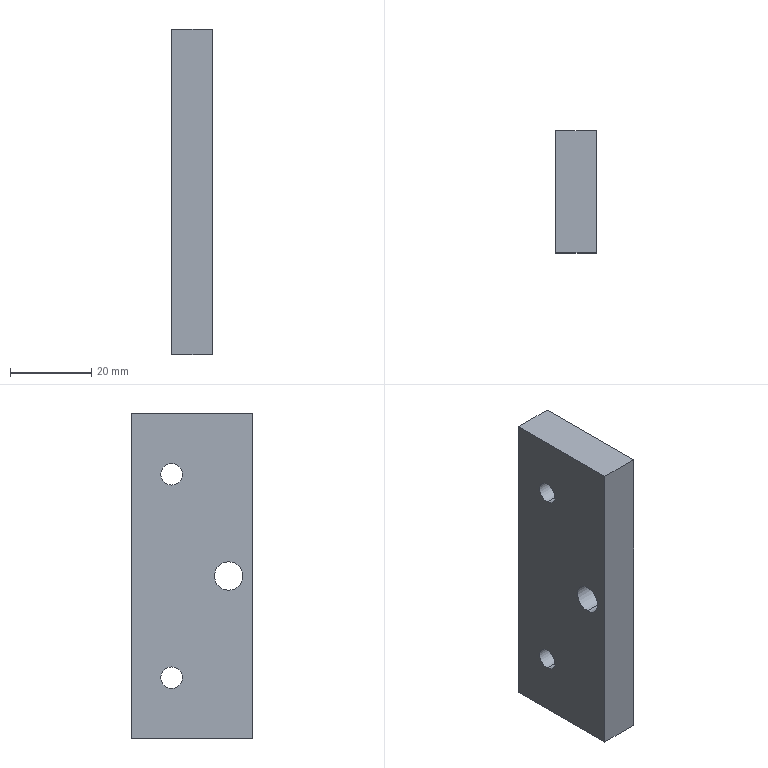Component | SolidWorks | A0131-1 | 1 solid | 18 faces | box 10 x 30 x 80 mm | volume 22564 mm3 | cylinder 10 | plane 8 | commonest cylinder face diameters 10 x4 5.3 x4 7 x2
build123d program:
from build123d import *

# Parameters (mm, degrees)
SKETCH1_W                                       = 80
SKETCH1_H                                       = 30
BOSS_EXTRUDE1_DEPTH                             = 10
M8X1_0_TAPPED_HOLE1_D                           = 7
M5_HEX_SOCKET_HEAD_CAP_SCREW_CBORE1_D           = 5.3
M5_HEX_SOCKET_HEAD_CAP_SCREW_CBORE1_CBORE_D     = 10
M5_HEX_SOCKET_HEAD_CAP_SCREW_CBORE1_CBORE_DEPTH = 5.4


with BuildPart() as part:
    # Sketch1 → Boss-Extrude1 (new body)
    with BuildSketch(Plane.XY):
        Rectangle(SKETCH1_W, SKETCH1_H)
    extrude(amount=BOSS_EXTRUDE1_DEPTH)

    # M8x1.0 Tapped Hole1 (through all)
    with Locations(Plane.XY.offset(10)):
        with Locations((0, 9)):
            Hole(M8X1_0_TAPPED_HOLE1_D / 2)

    # M5 Hex Socket Head Cap Screw CBORE1 (through all)
    with Locations(Plane.XY.offset(10)):
        with Locations((-25, -5), (25, -5)):
            CounterBoreHole(M5_HEX_SOCKET_HEAD_CAP_SCREW_CBORE1_D / 2, M5_HEX_SOCKET_HEAD_CAP_SCREW_CBORE1_CBORE_D / 2, M5_HEX_SOCKET_HEAD_CAP_SCREW_CBORE1_CBORE_DEPTH)


solid = part.part

# Placed as in the assembly
solid = solid.moved(Location((-38.619, 56, 60), (180, 90, 0)))
STEP:
#1=COLOUR_RGB('',0.7922,0.8196,0.9333);
#2=FILL_AREA_STYLE_COLOUR('',#1);
#3=FILL_AREA_STYLE('',(#2));
#4=SURFACE_STYLE_FILL_AREA(#3);
#5=SURFACE_SIDE_STYLE('',(#4));
#6=SURFACE_STYLE_USAGE(.BOTH.,#5);
#7=PRESENTATION_STYLE_ASSIGNMENT((#6));
#8=CARTESIAN_POINT('',(-1.339,2.402,1.181));
#9=VERTEX_POINT('',#8);
#10=CARTESIAN_POINT('',(-1.339,2.402,1.575));
#11=VERTEX_POINT('',#10);
#12=CARTESIAN_POINT('',(-1.339,2.402,1.378));
#13=DIRECTION('',(1.,-0.,-0.));
#14=DIRECTION('',(0.,0.,1.));
#15=AXIS2_PLACEMENT_3D('',#12,#13,#14);
#16=CIRCLE('',#15,0.1969);
#17=EDGE_CURVE('',#9,#11,#16,.T.);
#18=ORIENTED_EDGE('',*,*,#17,.F.);
#19=CARTESIAN_POINT('',(-1.127,2.402,1.181));
#20=VERTEX_POINT('',#19);
#21=CARTESIAN_POINT('',(-1.127,2.402,1.181));
#22=DIRECTION('',(1.,-0.,-0.));
#23=VECTOR('',#22,39.37);
#24=LINE('',#21,#23);
#25=EDGE_CURVE('',#9,#20,#24,.T.);
#26=ORIENTED_EDGE('',*,*,#25,.T.);
#27=CARTESIAN_POINT('',(-1.127,2.402,1.575));
#28=VERTEX_POINT('',#27);
#29=CARTESIAN_POINT('',(-1.127,2.402,1.378));
#30=DIRECTION('',(1.,-0.,-0.));
#31=DIRECTION('',(0.,0.,1.));
#32=AXIS2_PLACEMENT_3D('',#29,#30,#31);
#33=CIRCLE('',#32,0.1969);
#34=EDGE_CURVE('',#20,#28,#33,.T.);
#35=ORIENTED_EDGE('',*,*,#34,.T.);
#36=CARTESIAN_POINT('',(-1.127,2.402,1.575));
#37=DIRECTION('',(1.,-0.,-0.));
#38=VECTOR('',#37,39.37);
#39=LINE('',#36,#38);
#40=EDGE_CURVE('',#11,#28,#39,.T.);
#41=ORIENTED_EDGE('',*,*,#40,.F.);
#42=EDGE_LOOP('',(#18,#26,#35,#41));
#43=FACE_OUTER_BOUND('',#42,.T.);
#44=CARTESIAN_POINT('',(-1.127,2.402,1.378));
#45=DIRECTION('',(1.,-0.,-0.));
#46=DIRECTION('',(0.,0.,1.));
#47=AXIS2_PLACEMENT_3D('',#44,#45,#46);
#48=CYLINDRICAL_SURFACE('',#47,0.1969);
#49=ADVANCED_FACE('',(#43),#48,.F.);
#50=CARTESIAN_POINT('',(-1.52,2.402,1.274));
#51=VERTEX_POINT('',#50);
#52=CARTESIAN_POINT('',(-1.52,2.402,1.482));
#53=VERTEX_POINT('',#52);
#54=CARTESIAN_POINT('',(-1.52,2.402,1.378));
#55=DIRECTION('',(1.,-0.,-0.));
#56=DIRECTION('',(0.,0.,1.));
#57=AXIS2_PLACEMENT_3D('',#54,#55,#56);
#58=CIRCLE('',#57,0.1043);
#59=EDGE_CURVE('',#51,#53,#58,.T.);
#60=ORIENTED_EDGE('',*,*,#59,.F.);
#61=CARTESIAN_POINT('',(-1.339,2.402,1.274));
#62=VERTEX_POINT('',#61);
#63=CARTESIAN_POINT('',(-1.127,2.402,1.274));
#64=DIRECTION('',(1.,-0.,-0.));
#65=VECTOR('',#64,39.37);
#66=LINE('',#63,#65);
#67=EDGE_CURVE('',#51,#62,#66,.T.);
#68=ORIENTED_EDGE('',*,*,#67,.T.);
#69=CARTESIAN_POINT('',(-1.339,2.402,1.482));
#70=VERTEX_POINT('',#69);
#71=CARTESIAN_POINT('',(-1.339,2.402,1.378));
#72=DIRECTION('',(1.,-0.,-0.));
#73=DIRECTION('',(0.,0.,1.));
#74=AXIS2_PLACEMENT_3D('',#71,#72,#73);
#75=CIRCLE('',#74,0.1043);
#76=EDGE_CURVE('',#62,#70,#75,.T.);
#77=ORIENTED_EDGE('',*,*,#76,.T.);
#78=CARTESIAN_POINT('',(-1.127,2.402,1.482));
#79=DIRECTION('',(1.,-0.,-0.));
#80=VECTOR('',#79,39.37);
#81=LINE('',#78,#80);
#82=EDGE_CURVE('',#53,#70,#81,.T.);
#83=ORIENTED_EDGE('',*,*,#82,.F.);
#84=EDGE_LOOP('',(#60,#68,#77,#83));
#85=FACE_OUTER_BOUND('',#84,.T.);
#86=CARTESIAN_POINT('',(-1.127,2.402,1.378));
#87=DIRECTION('',(1.,-0.,-0.));
#88=DIRECTION('',(0.,0.,1.));
#89=AXIS2_PLACEMENT_3D('',#86,#87,#88);
#90=CYLINDRICAL_SURFACE('',#89,0.1043);
#91=ADVANCED_FACE('',(#85),#90,.F.);
#92=CARTESIAN_POINT('',(-1.339,2.402,3.15));
#93=VERTEX_POINT('',#92);
#94=CARTESIAN_POINT('',(-1.339,2.402,3.543));
#95=VERTEX_POINT('',#94);
#96=CARTESIAN_POINT('',(-1.339,2.402,3.346));
#97=DIRECTION('',(1.,-0.,-0.));
#98=DIRECTION('',(0.,0.,1.));
#99=AXIS2_PLACEMENT_3D('',#96,#97,#98);
#100=CIRCLE('',#99,0.1969);
#101=EDGE_CURVE('',#93,#95,#100,.T.);
#102=ORIENTED_EDGE('',*,*,#101,.F.);
#103=CARTESIAN_POINT('',(-1.127,2.402,3.15));
#104=VERTEX_POINT('',#103);
#105=CARTESIAN_POINT('',(-1.127,2.402,3.15));
#106=DIRECTION('',(1.,-0.,-0.));
#107=VECTOR('',#106,39.37);
#108=LINE('',#105,#107);
#109=EDGE_CURVE('',#93,#104,#108,.T.);
#110=ORIENTED_EDGE('',*,*,#109,.T.);
#111=CARTESIAN_POINT('',(-1.127,2.402,3.543));
#112=VERTEX_POINT('',#111);
#113=CARTESIAN_POINT('',(-1.127,2.402,3.346));
#114=DIRECTION('',(1.,-0.,-0.));
#115=DIRECTION('',(0.,0.,1.));
#116=AXIS2_PLACEMENT_3D('',#113,#114,#115);
#117=CIRCLE('',#116,0.1969);
#118=EDGE_CURVE('',#104,#112,#117,.T.);
#119=ORIENTED_EDGE('',*,*,#118,.T.);
#120=CARTESIAN_POINT('',(-1.127,2.402,3.543));
#121=DIRECTION('',(1.,-0.,-0.));
#122=VECTOR('',#121,39.37);
#123=LINE('',#120,#122);
#124=EDGE_CURVE('',#95,#112,#123,.T.);
#125=ORIENTED_EDGE('',*,*,#124,.F.);
#126=EDGE_LOOP('',(#102,#110,#119,#125));
#127=FACE_OUTER_BOUND('',#126,.T.);
#128=CARTESIAN_POINT('',(-1.127,2.402,3.346));
#129=DIRECTION('',(1.,-0.,-0.));
#130=DIRECTION('',(0.,0.,1.));
#131=AXIS2_PLACEMENT_3D('',#128,#129,#130);
#132=CYLINDRICAL_SURFACE('',#131,0.1969);
#133=ADVANCED_FACE('',(#127),#132,.F.);
#134=CARTESIAN_POINT('',(-1.52,2.402,3.242));
#135=VERTEX_POINT('',#134);
#136=CARTESIAN_POINT('',(-1.52,2.402,3.451));
#137=VERTEX_POINT('',#136);
#138=CARTESIAN_POINT('',(-1.52,2.402,3.346));
#139=DIRECTION('',(1.,-0.,-0.));
#140=DIRECTION('',(0.,0.,1.));
#141=AXIS2_PLACEMENT_3D('',#138,#139,#140);
#142=CIRCLE('',#141,0.1043);
#143=EDGE_CURVE('',#135,#137,#142,.T.);
#144=ORIENTED_EDGE('',*,*,#143,.F.);
#145=CARTESIAN_POINT('',(-1.339,2.402,3.242));
#146=VERTEX_POINT('',#145);
#147=CARTESIAN_POINT('',(-1.127,2.402,3.242));
#148=DIRECTION('',(1.,-0.,-0.));
#149=VECTOR('',#148,39.37);
#150=LINE('',#147,#149);
#151=EDGE_CURVE('',#135,#146,#150,.T.);
#152=ORIENTED_EDGE('',*,*,#151,.T.);
#153=CARTESIAN_POINT('',(-1.339,2.402,3.451));
#154=VERTEX_POINT('',#153);
#155=CARTESIAN_POINT('',(-1.339,2.402,3.346));
#156=DIRECTION('',(1.,-0.,-0.));
#157=DIRECTION('',(0.,0.,1.));
#158=AXIS2_PLACEMENT_3D('',#155,#156,#157);
#159=CIRCLE('',#158,0.1043);
#160=EDGE_CURVE('',#146,#154,#159,.T.);
#161=ORIENTED_EDGE('',*,*,#160,.T.);
#162=CARTESIAN_POINT('',(-1.127,2.402,3.451));
#163=DIRECTION('',(1.,-0.,-0.));
#164=VECTOR('',#163,39.37);
#165=LINE('',#162,#164);
#166=EDGE_CURVE('',#137,#154,#165,.T.);
#167=ORIENTED_EDGE('',*,*,#166,.F.);
#168=EDGE_LOOP('',(#144,#152,#161,#167));
#169=FACE_OUTER_BOUND('',#168,.T.);
#170=CARTESIAN_POINT('',(-1.127,2.402,3.346));
#171=DIRECTION('',(1.,-0.,-0.));
#172=DIRECTION('',(0.,0.,1.));
#173=AXIS2_PLACEMENT_3D('',#170,#171,#172);
#174=CYLINDRICAL_SURFACE('',#173,0.1043);
#175=ADVANCED_FACE('',(#169),#174,.F.);
#176=CARTESIAN_POINT('',(-1.52,1.85,2.224));
#177=VERTEX_POINT('',#176);
#178=CARTESIAN_POINT('',(-1.52,1.85,2.5));
#179=VERTEX_POINT('',#178);
#180=CARTESIAN_POINT('',(-1.52,1.85,2.362));
#181=DIRECTION('',(1.,-0.,-0.));
#182=DIRECTION('',(0.,0.,1.));
#183=AXIS2_PLACEMENT_3D('',#180,#181,#182);
#184=CIRCLE('',#183,0.1378);
#185=EDGE_CURVE('',#177,#179,#184,.T.);
#186=ORIENTED_EDGE('',*,*,#185,.F.);
#187=CARTESIAN_POINT('',(-1.127,1.85,2.224));
#188=VERTEX_POINT('',#187);
#189=CARTESIAN_POINT('',(-1.127,1.85,2.224));
#190=DIRECTION('',(1.,-0.,-0.));
#191=VECTOR('',#190,39.37);
#192=LINE('',#189,#191);
#193=EDGE_CURVE('',#177,#188,#192,.T.);
#194=ORIENTED_EDGE('',*,*,#193,.T.);
#195=CARTESIAN_POINT('',(-1.127,1.85,2.5));
#196=VERTEX_POINT('',#195);
#197=CARTESIAN_POINT('',(-1.127,1.85,2.362));
#198=DIRECTION('',(1.,-0.,-0.));
#199=DIRECTION('',(0.,0.,1.));
#200=AXIS2_PLACEMENT_3D('',#197,#198,#199);
#201=CIRCLE('',#200,0.1378);
#202=EDGE_CURVE('',#188,#196,#201,.T.);
#203=ORIENTED_EDGE('',*,*,#202,.T.);
#204=CARTESIAN_POINT('',(-1.127,1.85,2.5));
#205=DIRECTION('',(1.,-0.,-0.));
#206=VECTOR('',#205,39.37);
#207=LINE('',#204,#206);
#208=EDGE_CURVE('',#179,#196,#207,.T.);
#209=ORIENTED_EDGE('',*,*,#208,.F.);
#210=EDGE_LOOP('',(#186,#194,#203,#209));
#211=FACE_OUTER_BOUND('',#210,.T.);
#212=CARTESIAN_POINT('',(-1.127,1.85,2.362));
#213=DIRECTION('',(1.,-0.,-0.));
#214=DIRECTION('',(0.,0.,1.));
#215=AXIS2_PLACEMENT_3D('',#212,#213,#214);
#216=CYLINDRICAL_SURFACE('',#215,0.1378);
#217=ADVANCED_FACE('',(#211),#216,.F.);
#218=CARTESIAN_POINT('',(-1.52,2.795,3.937));
#219=VERTEX_POINT('',#218);
#220=CARTESIAN_POINT('',(-1.52,1.614,3.937));
#221=VERTEX_POINT('',#220);
#222=CARTESIAN_POINT('',(-1.52,1.614,3.937));
#223=DIRECTION('',(-0.,-1.,-0.));
#224=VECTOR('',#223,39.37);
#225=LINE('',#222,#224);
#226=EDGE_CURVE('',#219,#221,#225,.T.);
#227=ORIENTED_EDGE('',*,*,#226,.T.);
#228=CARTESIAN_POINT('',(-1.127,1.614,3.937));
#229=VERTEX_POINT('',#228);
#230=CARTESIAN_POINT('',(-1.127,1.614,3.937));
#231=DIRECTION('',(-1.,0.,0.));
#232=VECTOR('',#231,39.37);
#233=LINE('',#230,#232);
#234=EDGE_CURVE('',#229,#221,#233,.T.);
#235=ORIENTED_EDGE('',*,*,#234,.F.);
#236=CARTESIAN_POINT('',(-1.127,2.795,3.937));
#237=VERTEX_POINT('',#236);
#238=CARTESIAN_POINT('',(-1.127,1.614,3.937));
#239=DIRECTION('',(-0.,-1.,-0.));
#240=VECTOR('',#239,39.37);
#241=LINE('',#238,#240);
#242=EDGE_CURVE('',#237,#229,#241,.T.);
#243=ORIENTED_EDGE('',*,*,#242,.F.);
#244=CARTESIAN_POINT('',(-1.127,2.795,3.937));
#245=DIRECTION('',(-1.,0.,0.));
#246=VECTOR('',#245,39.37);
#247=LINE('',#244,#246);
#248=EDGE_CURVE('',#237,#219,#247,.T.);
#249=ORIENTED_EDGE('',*,*,#248,.T.);
#250=EDGE_LOOP('',(#227,#235,#243,#249));
#251=FACE_OUTER_BOUND('',#250,.T.);
#252=CARTESIAN_POINT('',(-1.127,1.614,3.937));
#253=DIRECTION('',(-0.,0.,-1.));
#254=DIRECTION('',(0.,1.,0.));
#255=AXIS2_PLACEMENT_3D('',#252,#253,#254);
#256=PLANE('',#255);
#257=ADVANCED_FACE('',(#251),#256,.F.);
#258=CARTESIAN_POINT('',(-1.52,1.614,0.7874));
#259=VERTEX_POINT('',#258);
#260=CARTESIAN_POINT('',(-1.52,1.614,0.7874));
#261=DIRECTION('',(-0.,-0.,-1.));
#262=VECTOR('',#261,39.37);
#263=LINE('',#260,#262);
#264=EDGE_CURVE('',#221,#259,#263,.T.);
#265=ORIENTED_EDGE('',*,*,#264,.T.);
#266=CARTESIAN_POINT('',(-1.127,1.614,0.7874));
#267=VERTEX_POINT('',#266);
#268=CARTESIAN_POINT('',(-1.127,1.614,0.7874));
#269=DIRECTION('',(-1.,0.,0.));
#270=VECTOR('',#269,39.37);
#271=LINE('',#268,#270);
#272=EDGE_CURVE('',#267,#259,#271,.T.);
#273=ORIENTED_EDGE('',*,*,#272,.F.);
#274=CARTESIAN_POINT('',(-1.127,1.614,0.7874));
#275=DIRECTION('',(-0.,-0.,-1.));
#276=VECTOR('',#275,39.37);
#277=LINE('',#274,#276);
#278=EDGE_CURVE('',#229,#267,#277,.T.);
#279=ORIENTED_EDGE('',*,*,#278,.F.);
#280=ORIENTED_EDGE('',*,*,#234,.T.);
#281=EDGE_LOOP('',(#265,#273,#279,#280));
#282=FACE_OUTER_BOUND('',#281,.T.);
#283=CARTESIAN_POINT('',(-1.127,1.614,0.7874));
#284=DIRECTION('',(0.,1.,0.));
#285=DIRECTION('',(-1.,0.,0.));
#286=AXIS2_PLACEMENT_3D('',#283,#284,#285);
#287=PLANE('',#286);
#288=ADVANCED_FACE('',(#282),#287,.F.);
#289=CARTESIAN_POINT('',(-1.52,2.795,0.7874));
#290=VERTEX_POINT('',#289);
#291=CARTESIAN_POINT('',(-1.52,1.614,0.7874));
#292=DIRECTION('',(0.,1.,0.));
#293=VECTOR('',#292,39.37);
#294=LINE('',#291,#293);
#295=EDGE_CURVE('',#259,#290,#294,.T.);
#296=ORIENTED_EDGE('',*,*,#295,.T.);
#297=CARTESIAN_POINT('',(-1.127,2.795,0.7874));
#298=VERTEX_POINT('',#297);
#299=CARTESIAN_POINT('',(-1.127,2.795,0.7874));
#300=DIRECTION('',(-1.,0.,0.));
#301=VECTOR('',#300,39.37);
#302=LINE('',#299,#301);
#303=EDGE_CURVE('',#298,#290,#302,.T.);
#304=ORIENTED_EDGE('',*,*,#303,.F.);
#305=CARTESIAN_POINT('',(-1.127,1.614,0.7874));
#306=DIRECTION('',(0.,1.,0.));
#307=VECTOR('',#306,39.37);
#308=LINE('',#305,#307);
#309=EDGE_CURVE('',#267,#298,#308,.T.);
#310=ORIENTED_EDGE('',*,*,#309,.F.);
#311=ORIENTED_EDGE('',*,*,#272,.T.);
#312=EDGE_LOOP('',(#296,#304,#310,#311));
#313=FACE_OUTER_BOUND('',#312,.T.);
#314=CARTESIAN_POINT('',(-1.127,1.614,0.7874));
#315=DIRECTION('',(0.,0.,1.));
#316=DIRECTION('',(-1.,0.,0.));
#317=AXIS2_PLACEMENT_3D('',#314,#315,#316);
#318=PLANE('',#317);
#319=ADVANCED_FACE('',(#313),#318,.F.);
#320=CARTESIAN_POINT('',(-1.52,2.795,0.7874));
#321=DIRECTION('',(0.,0.,1.));
#322=VECTOR('',#321,39.37);
#323=LINE('',#320,#322);
#324=EDGE_CURVE('',#290,#219,#323,.T.);
#325=ORIENTED_EDGE('',*,*,#324,.T.);
#326=ORIENTED_EDGE('',*,*,#248,.F.);
#327=CARTESIAN_POINT('',(-1.127,2.795,0.7874));
#328=DIRECTION('',(0.,0.,1.));
#329=VECTOR('',#328,39.37);
#330=LINE('',#327,#329);
#331=EDGE_CURVE('',#298,#237,#330,.T.);
#332=ORIENTED_EDGE('',*,*,#331,.F.);
#333=ORIENTED_EDGE('',*,*,#303,.T.);
#334=EDGE_LOOP('',(#325,#326,#332,#333));
#335=FACE_OUTER_BOUND('',#334,.T.);
#336=CARTESIAN_POINT('',(-1.127,2.795,0.7874));
#337=DIRECTION('',(-0.,-1.,-0.));
#338=DIRECTION('',(1.,-0.,-0.));
#339=AXIS2_PLACEMENT_3D('',#336,#337,#338);
#340=PLANE('',#339);
#341=ADVANCED_FACE('',(#335),#340,.F.);
#342=CARTESIAN_POINT('',(-1.127,2.402,1.378));
#343=DIRECTION('',(1.,-0.,-0.));
#344=DIRECTION('',(0.,0.,1.));
#345=AXIS2_PLACEMENT_3D('',#342,#343,#344);
#346=CIRCLE('',#345,0.1969);
#347=EDGE_CURVE('',#28,#20,#346,.T.);
#348=ORIENTED_EDGE('',*,*,#347,.F.);
#349=ORIENTED_EDGE('',*,*,#34,.F.);
#350=EDGE_LOOP('',(#348,#349));
#351=FACE_BOUND('',#350,.T.);
#352=CARTESIAN_POINT('',(-1.127,2.402,3.346));
#353=DIRECTION('',(1.,-0.,-0.));
#354=DIRECTION('',(0.,0.,1.));
#355=AXIS2_PLACEMENT_3D('',#352,#353,#354);
#356=CIRCLE('',#355,0.1969);
#357=EDGE_CURVE('',#112,#104,#356,.T.);
#358=ORIENTED_EDGE('',*,*,#357,.F.);
#359=ORIENTED_EDGE('',*,*,#118,.F.);
#360=EDGE_LOOP('',(#358,#359));
#361=FACE_BOUND('',#360,.T.);
#362=CARTESIAN_POINT('',(-1.127,1.85,2.362));
#363=DIRECTION('',(1.,-0.,-0.));
#364=DIRECTION('',(0.,0.,1.));
#365=AXIS2_PLACEMENT_3D('',#362,#363,#364);
#366=CIRCLE('',#365,0.1378);
#367=EDGE_CURVE('',#196,#188,#366,.T.);
#368=ORIENTED_EDGE('',*,*,#367,.F.);
#369=ORIENTED_EDGE('',*,*,#202,.F.);
#370=EDGE_LOOP('',(#368,#369));
#371=FACE_BOUND('',#370,.T.);
#372=ORIENTED_EDGE('',*,*,#242,.T.);
#373=ORIENTED_EDGE('',*,*,#278,.T.);
#374=ORIENTED_EDGE('',*,*,#309,.T.);
#375=ORIENTED_EDGE('',*,*,#331,.T.);
#376=EDGE_LOOP('',(#372,#373,#374,#375));
#377=FACE_OUTER_BOUND('',#376,.T.);
#378=CARTESIAN_POINT('',(-1.127,2.205,2.362));
#379=DIRECTION('',(1.,-0.,-0.));
#380=DIRECTION('',(0.,0.,1.));
#381=AXIS2_PLACEMENT_3D('',#378,#379,#380);
#382=PLANE('',#381);
#383=ADVANCED_FACE('',(#351,#361,#371,#377),#382,.T.);
#384=CARTESIAN_POINT('',(-1.52,2.402,1.378));
#385=DIRECTION('',(1.,-0.,-0.));
#386=DIRECTION('',(0.,0.,1.));
#387=AXIS2_PLACEMENT_3D('',#384,#385,#386);
#388=CIRCLE('',#387,0.1043);
#389=EDGE_CURVE('',#53,#51,#388,.T.);
#390=ORIENTED_EDGE('',*,*,#389,.T.);
#391=ORIENTED_EDGE('',*,*,#59,.T.);
#392=EDGE_LOOP('',(#390,#391));
#393=FACE_BOUND('',#392,.T.);
#394=CARTESIAN_POINT('',(-1.52,2.402,3.346));
#395=DIRECTION('',(1.,-0.,-0.));
#396=DIRECTION('',(0.,0.,1.));
#397=AXIS2_PLACEMENT_3D('',#394,#395,#396);
#398=CIRCLE('',#397,0.1043);
#399=EDGE_CURVE('',#137,#135,#398,.T.);
#400=ORIENTED_EDGE('',*,*,#399,.T.);
#401=ORIENTED_EDGE('',*,*,#143,.T.);
#402=EDGE_LOOP('',(#400,#401));
#403=FACE_BOUND('',#402,.T.);
#404=CARTESIAN_POINT('',(-1.52,1.85,2.362));
#405=DIRECTION('',(1.,-0.,-0.));
#406=DIRECTION('',(0.,0.,1.));
#407=AXIS2_PLACEMENT_3D('',#404,#405,#406);
#408=CIRCLE('',#407,0.1378);
#409=EDGE_CURVE('',#179,#177,#408,.T.);
#410=ORIENTED_EDGE('',*,*,#409,.T.);
#411=ORIENTED_EDGE('',*,*,#185,.T.);
#412=EDGE_LOOP('',(#410,#411));
#413=FACE_BOUND('',#412,.T.);
#414=ORIENTED_EDGE('',*,*,#226,.F.);
#415=ORIENTED_EDGE('',*,*,#324,.F.);
#416=ORIENTED_EDGE('',*,*,#295,.F.);
#417=ORIENTED_EDGE('',*,*,#264,.F.);
#418=EDGE_LOOP('',(#414,#415,#416,#417));
#419=FACE_OUTER_BOUND('',#418,.T.);
#420=CARTESIAN_POINT('',(-1.52,2.205,2.362));
#421=DIRECTION('',(1.,-0.,-0.));
#422=DIRECTION('',(0.,0.,1.));
#423=AXIS2_PLACEMENT_3D('',#420,#421,#422);
#424=PLANE('',#423);
#425=ADVANCED_FACE('',(#393,#403,#413,#419),#424,.F.);
#426=ORIENTED_EDGE('',*,*,#193,.F.);
#427=ORIENTED_EDGE('',*,*,#409,.F.);
#428=ORIENTED_EDGE('',*,*,#208,.T.);
#429=ORIENTED_EDGE('',*,*,#367,.T.);
#430=EDGE_LOOP('',(#426,#427,#428,#429));
#431=FACE_OUTER_BOUND('',#430,.T.);
#432=CARTESIAN_POINT('',(-1.127,1.85,2.362));
#433=DIRECTION('',(1.,-0.,-0.));
#434=DIRECTION('',(0.,0.,1.));
#435=AXIS2_PLACEMENT_3D('',#432,#433,#434);
#436=CYLINDRICAL_SURFACE('',#435,0.1378);
#437=ADVANCED_FACE('',(#431),#436,.F.);
#438=ORIENTED_EDGE('',*,*,#151,.F.);
#439=ORIENTED_EDGE('',*,*,#399,.F.);
#440=ORIENTED_EDGE('',*,*,#166,.T.);
#441=CARTESIAN_POINT('',(-1.339,2.402,3.346));
#442=DIRECTION('',(1.,-0.,-0.));
#443=DIRECTION('',(0.,0.,1.));
#444=AXIS2_PLACEMENT_3D('',#441,#442,#443);
#445=CIRCLE('',#444,0.1043);
#446=EDGE_CURVE('',#154,#146,#445,.T.);
#447=ORIENTED_EDGE('',*,*,#446,.T.);
#448=EDGE_LOOP('',(#438,#439,#440,#447));
#449=FACE_OUTER_BOUND('',#448,.T.);
#450=CARTESIAN_POINT('',(-1.127,2.402,3.346));
#451=DIRECTION('',(1.,-0.,-0.));
#452=DIRECTION('',(0.,0.,1.));
#453=AXIS2_PLACEMENT_3D('',#450,#451,#452);
#454=CYLINDRICAL_SURFACE('',#453,0.1043);
#455=ADVANCED_FACE('',(#449),#454,.F.);
#456=ORIENTED_EDGE('',*,*,#446,.F.);
#457=ORIENTED_EDGE('',*,*,#160,.F.);
#458=EDGE_LOOP('',(#456,#457));
#459=FACE_BOUND('',#458,.T.);
#460=CARTESIAN_POINT('',(-1.339,2.402,3.346));
#461=DIRECTION('',(1.,-0.,-0.));
#462=DIRECTION('',(0.,0.,1.));
#463=AXIS2_PLACEMENT_3D('',#460,#461,#462);
#464=CIRCLE('',#463,0.1969);
#465=EDGE_CURVE('',#95,#93,#464,.T.);
#466=ORIENTED_EDGE('',*,*,#465,.T.);
#467=ORIENTED_EDGE('',*,*,#101,.T.);
#468=EDGE_LOOP('',(#466,#467));
#469=FACE_OUTER_BOUND('',#468,.T.);
#470=CARTESIAN_POINT('',(-1.339,2.402,3.451));
#471=DIRECTION('',(-1.,0.,0.));
#472=DIRECTION('',(-0.,-0.,-1.));
#473=AXIS2_PLACEMENT_3D('',#470,#471,#472);
#474=PLANE('',#473);
#475=ADVANCED_FACE('',(#459,#469),#474,.F.);
#476=ORIENTED_EDGE('',*,*,#109,.F.);
#477=ORIENTED_EDGE('',*,*,#465,.F.);
#478=ORIENTED_EDGE('',*,*,#124,.T.);
#479=ORIENTED_EDGE('',*,*,#357,.T.);
#480=EDGE_LOOP('',(#476,#477,#478,#479));
#481=FACE_OUTER_BOUND('',#480,.T.);
#482=CARTESIAN_POINT('',(-1.127,2.402,3.346));
#483=DIRECTION('',(1.,-0.,-0.));
#484=DIRECTION('',(0.,0.,1.));
#485=AXIS2_PLACEMENT_3D('',#482,#483,#484);
#486=CYLINDRICAL_SURFACE('',#485,0.1969);
#487=ADVANCED_FACE('',(#481),#486,.F.);
#488=ORIENTED_EDGE('',*,*,#67,.F.);
#489=ORIENTED_EDGE('',*,*,#389,.F.);
#490=ORIENTED_EDGE('',*,*,#82,.T.);
#491=CARTESIAN_POINT('',(-1.339,2.402,1.378));
#492=DIRECTION('',(1.,-0.,-0.));
#493=DIRECTION('',(0.,0.,1.));
#494=AXIS2_PLACEMENT_3D('',#491,#492,#493);
#495=CIRCLE('',#494,0.1043);
#496=EDGE_CURVE('',#70,#62,#495,.T.);
#497=ORIENTED_EDGE('',*,*,#496,.T.);
#498=EDGE_LOOP('',(#488,#489,#490,#497));
#499=FACE_OUTER_BOUND('',#498,.T.);
#500=CARTESIAN_POINT('',(-1.127,2.402,1.378));
#501=DIRECTION('',(1.,-0.,-0.));
#502=DIRECTION('',(0.,0.,1.));
#503=AXIS2_PLACEMENT_3D('',#500,#501,#502);
#504=CYLINDRICAL_SURFACE('',#503,0.1043);
#505=ADVANCED_FACE('',(#499),#504,.F.);
#506=ORIENTED_EDGE('',*,*,#496,.F.);
#507=ORIENTED_EDGE('',*,*,#76,.F.);
#508=EDGE_LOOP('',(#506,#507));
#509=FACE_BOUND('',#508,.T.);
#510=CARTESIAN_POINT('',(-1.339,2.402,1.378));
#511=DIRECTION('',(1.,-0.,-0.));
#512=DIRECTION('',(0.,0.,1.));
#513=AXIS2_PLACEMENT_3D('',#510,#511,#512);
#514=CIRCLE('',#513,0.1969);
#515=EDGE_CURVE('',#11,#9,#514,.T.);
#516=ORIENTED_EDGE('',*,*,#515,.T.);
#517=ORIENTED_EDGE('',*,*,#17,.T.);
#518=EDGE_LOOP('',(#516,#517));
#519=FACE_OUTER_BOUND('',#518,.T.);
#520=CARTESIAN_POINT('',(-1.339,2.402,1.482));
#521=DIRECTION('',(-1.,0.,0.));
#522=DIRECTION('',(-0.,-0.,-1.));
#523=AXIS2_PLACEMENT_3D('',#520,#521,#522);
#524=PLANE('',#523);
#525=ADVANCED_FACE('',(#509,#519),#524,.F.);
#526=ORIENTED_EDGE('',*,*,#25,.F.);
#527=ORIENTED_EDGE('',*,*,#515,.F.);
#528=ORIENTED_EDGE('',*,*,#40,.T.);
#529=ORIENTED_EDGE('',*,*,#347,.T.);
#530=EDGE_LOOP('',(#526,#527,#528,#529));
#531=FACE_OUTER_BOUND('',#530,.T.);
#532=CARTESIAN_POINT('',(-1.127,2.402,1.378));
#533=DIRECTION('',(1.,-0.,-0.));
#534=DIRECTION('',(0.,0.,1.));
#535=AXIS2_PLACEMENT_3D('',#532,#533,#534);
#536=CYLINDRICAL_SURFACE('',#535,0.1969);
#537=ADVANCED_FACE('',(#531),#536,.F.);
#538=CLOSED_SHELL('',(#49,#91,#133,#175,#217,#257,#288,#319,#341,#383,#425,#437,#455,#475,#487,#505,#525,#537));
#539=MANIFOLD_SOLID_BREP('',#538);
#540=STYLED_ITEM('',(#7),#539);
#541=PRESENTATION_LAYER_ASSIGNMENT('','',(#540));
#542=(LENGTH_UNIT()NAMED_UNIT(*)SI_UNIT($,.METRE.));
#543=LENGTH_MEASURE_WITH_UNIT(LENGTH_MEASURE(0.0254),#542);
#544=DIMENSIONAL_EXPONENTS(1.,0.,0.,0.,0.,0.,0.);
#545=(CONVERSION_BASED_UNIT('',#543)LENGTH_UNIT()NAMED_UNIT(#544));
#546=UNCERTAINTY_MEASURE_WITH_UNIT(LENGTH_MEASURE(0.00001),#545,'','');
#547=(NAMED_UNIT(*)PLANE_ANGLE_UNIT()SI_UNIT($,.RADIAN.));
#548=(NAMED_UNIT(*)SI_UNIT($,.STERADIAN.)SOLID_ANGLE_UNIT());
#549=(GEOMETRIC_REPRESENTATION_CONTEXT(3)GLOBAL_UNCERTAINTY_ASSIGNED_CONTEXT((#546))GLOBAL_UNIT_ASSIGNED_CONTEXT((#545,#547,#548))REPRESENTATION_CONTEXT('',''));
#550=MECHANICAL_DESIGN_GEOMETRIC_PRESENTATION_REPRESENTATION('',(#540),#549);
#551=CARTESIAN_POINT('',(0.,0.,0.));
#552=DIRECTION('',(0.,0.,1.));
#553=DIRECTION('',(1.,0.,0.));
#554=AXIS2_PLACEMENT_3D('',#551,#552,#553);
#555=(LENGTH_UNIT()NAMED_UNIT(*)SI_UNIT($,.METRE.));
#556=LENGTH_MEASURE_WITH_UNIT(LENGTH_MEASURE(0.0254),#555);
#557=DIMENSIONAL_EXPONENTS(1.,0.,0.,0.,0.,0.,0.);
#558=(CONVERSION_BASED_UNIT('',#556)LENGTH_UNIT()NAMED_UNIT(#557));
#559=UNCERTAINTY_MEASURE_WITH_UNIT(LENGTH_MEASURE(0.00001),#558,'','');
#560=(NAMED_UNIT(*)PLANE_ANGLE_UNIT()SI_UNIT($,.RADIAN.));
#561=(NAMED_UNIT(*)SI_UNIT($,.STERADIAN.)SOLID_ANGLE_UNIT());
#562=(GEOMETRIC_REPRESENTATION_CONTEXT(3)GLOBAL_UNCERTAINTY_ASSIGNED_CONTEXT((#559))GLOBAL_UNIT_ASSIGNED_CONTEXT((#558,#560,#561))REPRESENTATION_CONTEXT('',''));
#563=ADVANCED_BREP_SHAPE_REPRESENTATION('',(#539,#554),#562);